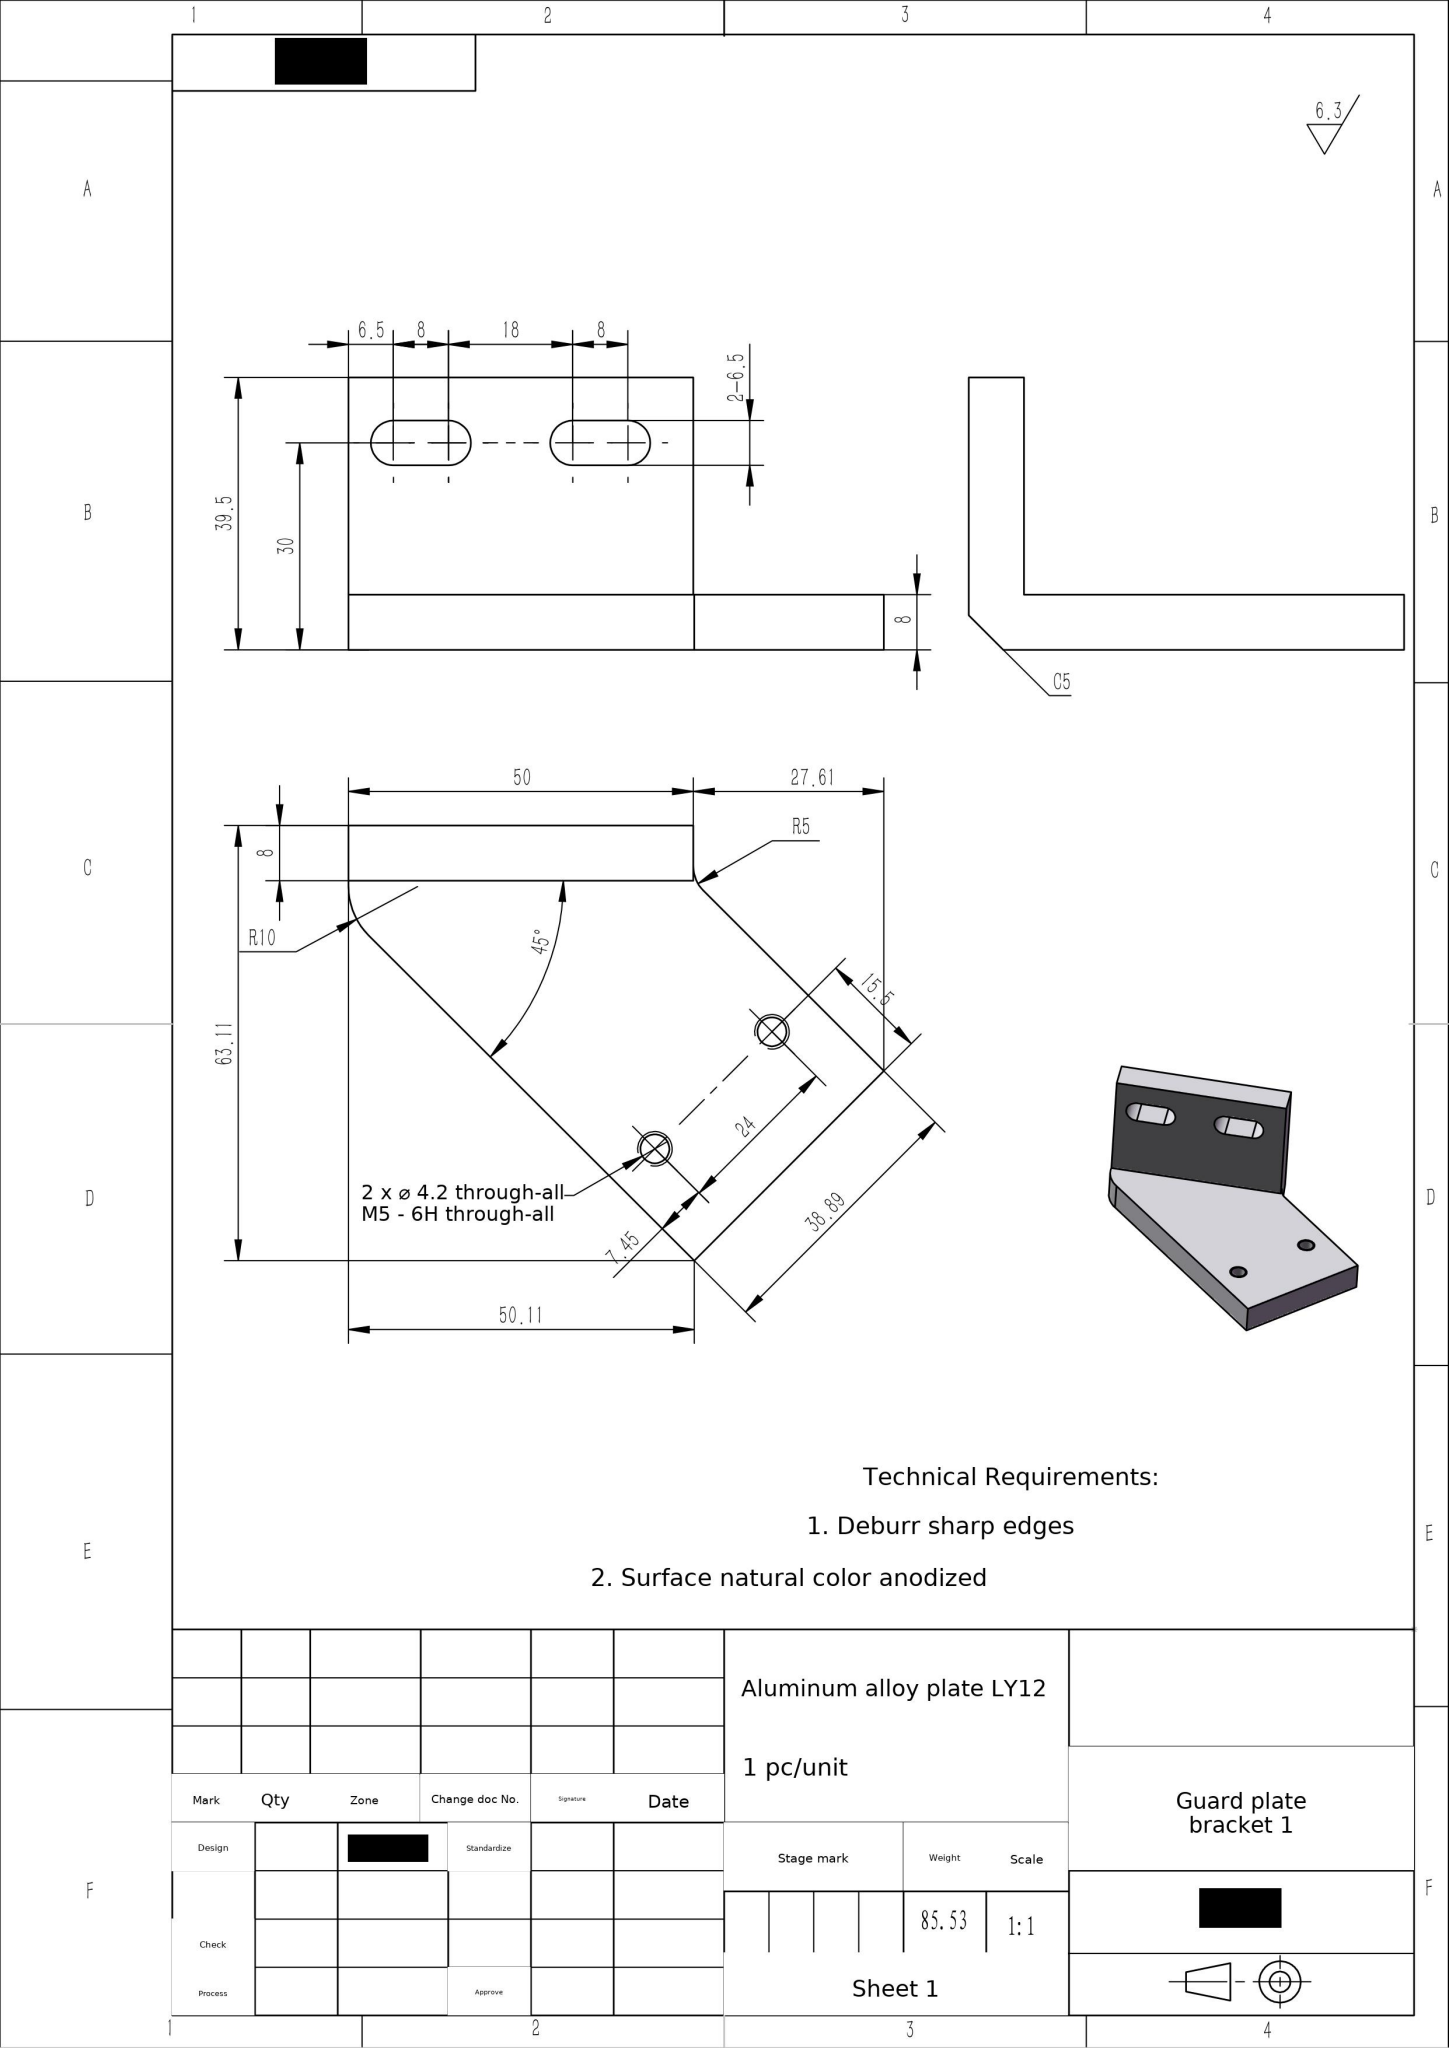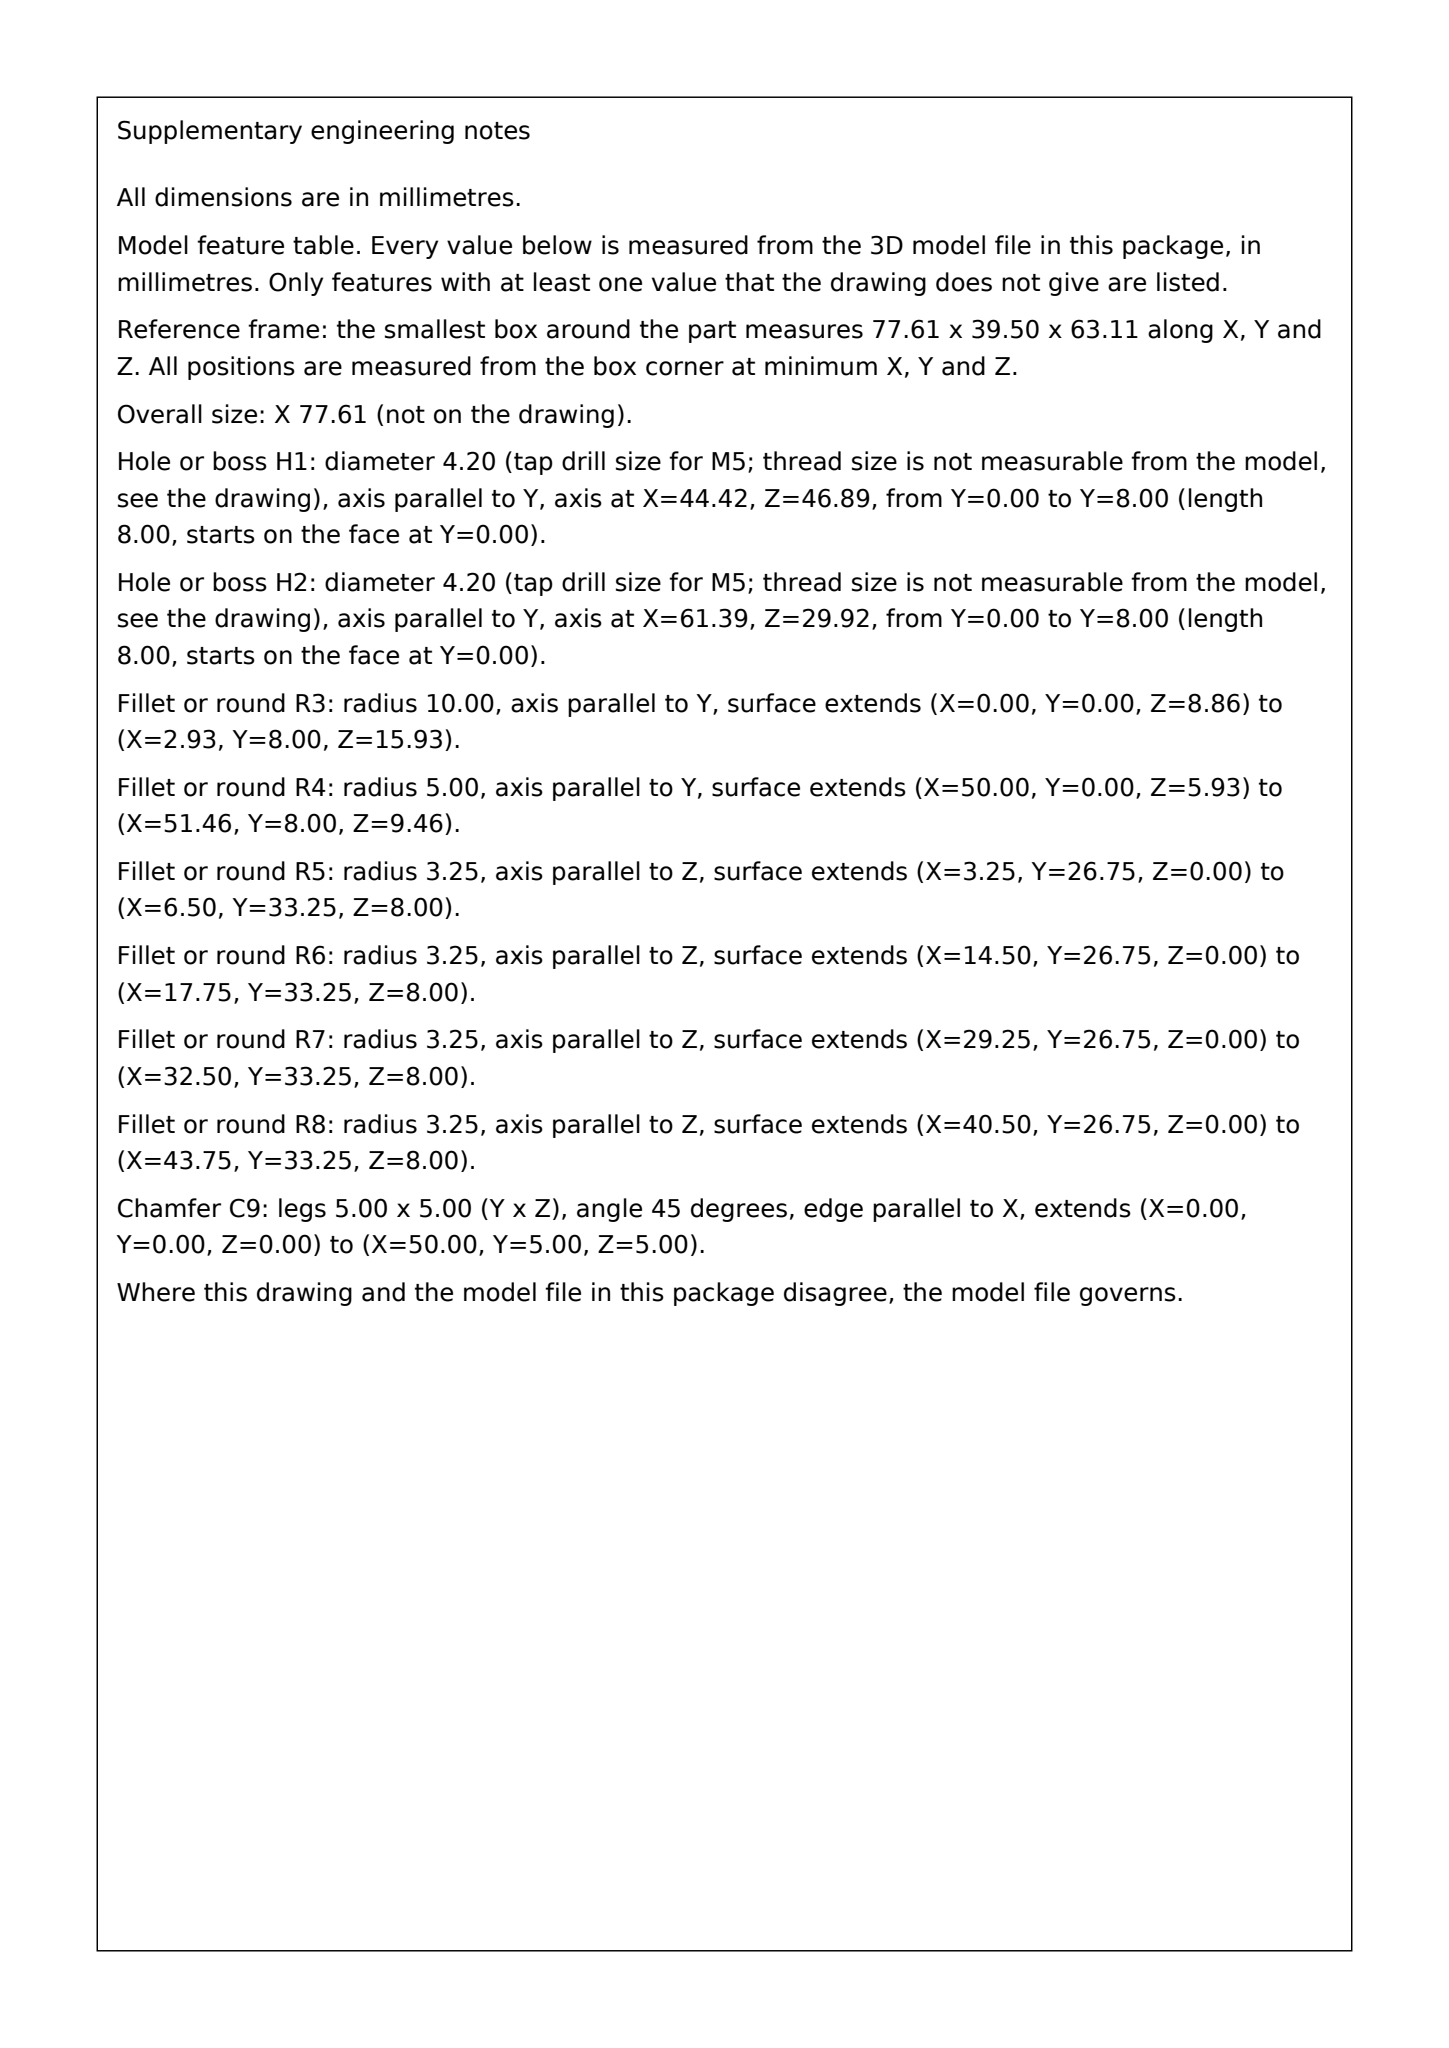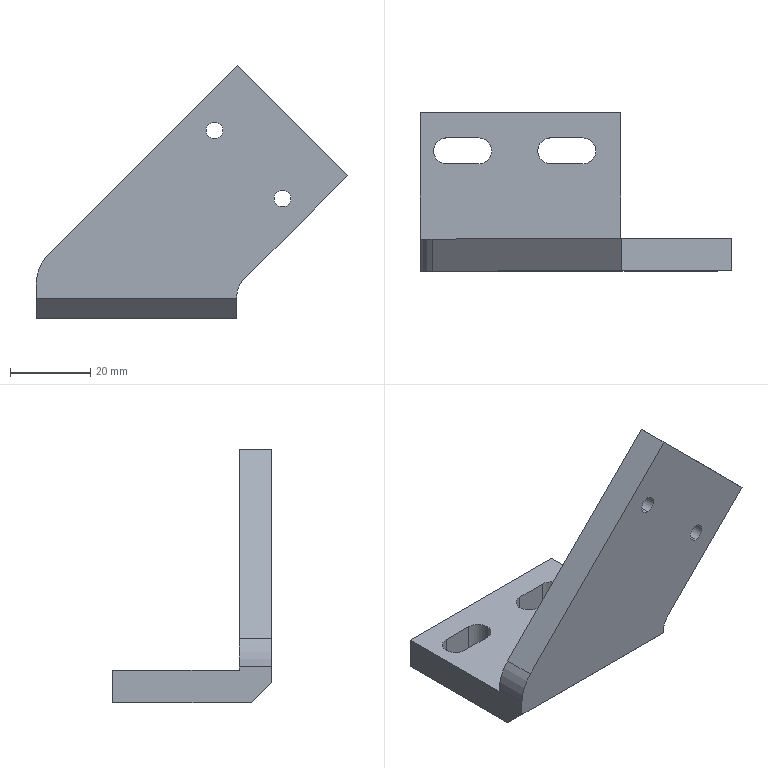Part | SolidWorks | mm | material Aluminum alloy plate LY12 | 1 solid | 27 faces | box 77.61 x 39.5 x 63.11 mm | volume 31677 mm3 | plane 15 | cylinder 12 | commonest cylinder face diameters 6.5 x6 4.2 x4 10 x1 20 x1
STEP:
#1=CARTESIAN_POINT('',(38.887,-24.,27.816));
#2=VERTEX_POINT('',#1);
#3=CARTESIAN_POINT('',(38.887,-24.,32.016));
#4=VERTEX_POINT('',#3);
#5=CARTESIAN_POINT('',(38.887,-24.,29.916));
#6=DIRECTION('',(0.,1.,0.));
#7=DIRECTION('',(0.,0.,1.));
#8=AXIS2_PLACEMENT_3D('',#5,#6,#7);
#9=CIRCLE('',#8,2.1);
#10=EDGE_CURVE('',#2,#4,#9,.T.);
#11=ORIENTED_EDGE('',*,*,#10,.F.);
#12=CARTESIAN_POINT('',(38.887,-16.,27.816));
#13=VERTEX_POINT('',#12);
#14=CARTESIAN_POINT('',(38.887,-16.,27.816));
#15=DIRECTION('',(0.,1.,0.));
#16=VECTOR('',#15,1000.);
#17=LINE('',#14,#16);
#18=EDGE_CURVE('',#2,#13,#17,.T.);
#19=ORIENTED_EDGE('',*,*,#18,.T.);
#20=CARTESIAN_POINT('',(38.887,-16.,32.016));
#21=VERTEX_POINT('',#20);
#22=CARTESIAN_POINT('',(38.887,-16.,29.916));
#23=DIRECTION('',(0.,1.,0.));
#24=DIRECTION('',(0.,0.,1.));
#25=AXIS2_PLACEMENT_3D('',#22,#23,#24);
#26=CIRCLE('',#25,2.1);
#27=EDGE_CURVE('',#13,#21,#26,.T.);
#28=ORIENTED_EDGE('',*,*,#27,.T.);
#29=CARTESIAN_POINT('',(38.887,-16.,32.016));
#30=DIRECTION('',(0.,1.,0.));
#31=VECTOR('',#30,1000.);
#32=LINE('',#29,#31);
#33=EDGE_CURVE('',#4,#21,#32,.T.);
#34=ORIENTED_EDGE('',*,*,#33,.F.);
#35=EDGE_LOOP('',(#11,#19,#28,#34));
#36=FACE_OUTER_BOUND('',#35,.T.);
#37=CARTESIAN_POINT('',(38.887,-16.,29.916));
#38=DIRECTION('',(0.,1.,0.));
#39=DIRECTION('',(0.,0.,1.));
#40=AXIS2_PLACEMENT_3D('',#37,#38,#39);
#41=CYLINDRICAL_SURFACE('',#40,2.1);
#42=ADVANCED_FACE('',(#36),#41,.F.);
#43=CARTESIAN_POINT('',(21.916,-24.,44.787));
#44=VERTEX_POINT('',#43);
#45=CARTESIAN_POINT('',(21.916,-24.,48.987));
#46=VERTEX_POINT('',#45);
#47=CARTESIAN_POINT('',(21.916,-24.,46.887));
#48=DIRECTION('',(0.,1.,0.));
#49=DIRECTION('',(0.,0.,1.));
#50=AXIS2_PLACEMENT_3D('',#47,#48,#49);
#51=CIRCLE('',#50,2.1);
#52=EDGE_CURVE('',#44,#46,#51,.T.);
#53=ORIENTED_EDGE('',*,*,#52,.F.);
#54=CARTESIAN_POINT('',(21.916,-16.,44.787));
#55=VERTEX_POINT('',#54);
#56=CARTESIAN_POINT('',(21.916,-16.,44.787));
#57=DIRECTION('',(0.,1.,0.));
#58=VECTOR('',#57,1000.);
#59=LINE('',#56,#58);
#60=EDGE_CURVE('',#44,#55,#59,.T.);
#61=ORIENTED_EDGE('',*,*,#60,.T.);
#62=CARTESIAN_POINT('',(21.916,-16.,48.987));
#63=VERTEX_POINT('',#62);
#64=CARTESIAN_POINT('',(21.916,-16.,46.887));
#65=DIRECTION('',(0.,1.,0.));
#66=DIRECTION('',(0.,0.,1.));
#67=AXIS2_PLACEMENT_3D('',#64,#65,#66);
#68=CIRCLE('',#67,2.1);
#69=EDGE_CURVE('',#55,#63,#68,.T.);
#70=ORIENTED_EDGE('',*,*,#69,.T.);
#71=CARTESIAN_POINT('',(21.916,-16.,48.987));
#72=DIRECTION('',(0.,1.,0.));
#73=VECTOR('',#72,1000.);
#74=LINE('',#71,#73);
#75=EDGE_CURVE('',#46,#63,#74,.T.);
#76=ORIENTED_EDGE('',*,*,#75,.F.);
#77=EDGE_LOOP('',(#53,#61,#70,#76));
#78=FACE_OUTER_BOUND('',#77,.T.);
#79=CARTESIAN_POINT('',(21.916,-16.,46.887));
#80=DIRECTION('',(0.,1.,0.));
#81=DIRECTION('',(0.,0.,1.));
#82=AXIS2_PLACEMENT_3D('',#79,#80,#81);
#83=CYLINDRICAL_SURFACE('',#82,2.1);
#84=ADVANCED_FACE('',(#78),#83,.F.);
#85=CARTESIAN_POINT('',(-4.75,6.,0.));
#86=VERTEX_POINT('',#85);
#87=CARTESIAN_POINT('',(-8.,9.25,0.));
#88=VERTEX_POINT('',#87);
#89=CARTESIAN_POINT('',(-8.,6.,0.));
#90=DIRECTION('',(0.,0.,1.));
#91=DIRECTION('',(1.,0.,0.));
#92=AXIS2_PLACEMENT_3D('',#89,#90,#91);
#93=CIRCLE('',#92,3.25);
#94=EDGE_CURVE('',#86,#88,#93,.T.);
#95=ORIENTED_EDGE('',*,*,#94,.F.);
#96=CARTESIAN_POINT('',(-4.75,6.,8.));
#97=VERTEX_POINT('',#96);
#98=CARTESIAN_POINT('',(-4.75,6.,0.));
#99=DIRECTION('',(0.,0.,1.));
#100=VECTOR('',#99,1000.);
#101=LINE('',#98,#100);
#102=EDGE_CURVE('',#86,#97,#101,.T.);
#103=ORIENTED_EDGE('',*,*,#102,.T.);
#104=CARTESIAN_POINT('',(-8.,9.25,8.));
#105=VERTEX_POINT('',#104);
#106=CARTESIAN_POINT('',(-8.,6.,8.));
#107=DIRECTION('',(0.,0.,1.));
#108=DIRECTION('',(1.,0.,0.));
#109=AXIS2_PLACEMENT_3D('',#106,#107,#108);
#110=CIRCLE('',#109,3.25);
#111=EDGE_CURVE('',#97,#105,#110,.T.);
#112=ORIENTED_EDGE('',*,*,#111,.T.);
#113=CARTESIAN_POINT('',(-8.,9.25,0.));
#114=DIRECTION('',(0.,0.,1.));
#115=VECTOR('',#114,1000.);
#116=LINE('',#113,#115);
#117=EDGE_CURVE('',#88,#105,#116,.T.);
#118=ORIENTED_EDGE('',*,*,#117,.F.);
#119=EDGE_LOOP('',(#95,#103,#112,#118));
#120=FACE_OUTER_BOUND('',#119,.T.);
#121=CARTESIAN_POINT('',(-8.,6.,0.));
#122=DIRECTION('',(0.,0.,1.));
#123=DIRECTION('',(1.,0.,0.));
#124=AXIS2_PLACEMENT_3D('',#121,#122,#123);
#125=CYLINDRICAL_SURFACE('',#124,3.25);
#126=ADVANCED_FACE('',(#120),#125,.F.);
#127=CARTESIAN_POINT('',(21.25,6.,0.));
#128=VERTEX_POINT('',#127);
#129=CARTESIAN_POINT('',(18.,9.25,0.));
#130=VERTEX_POINT('',#129);
#131=CARTESIAN_POINT('',(18.,6.,0.));
#132=DIRECTION('',(0.,0.,1.));
#133=DIRECTION('',(-1.,0.,0.));
#134=AXIS2_PLACEMENT_3D('',#131,#132,#133);
#135=CIRCLE('',#134,3.25);
#136=EDGE_CURVE('',#128,#130,#135,.T.);
#137=ORIENTED_EDGE('',*,*,#136,.F.);
#138=CARTESIAN_POINT('',(21.25,6.,8.));
#139=VERTEX_POINT('',#138);
#140=CARTESIAN_POINT('',(21.25,6.,0.));
#141=DIRECTION('',(0.,0.,1.));
#142=VECTOR('',#141,1000.);
#143=LINE('',#140,#142);
#144=EDGE_CURVE('',#128,#139,#143,.T.);
#145=ORIENTED_EDGE('',*,*,#144,.T.);
#146=CARTESIAN_POINT('',(18.,9.25,8.));
#147=VERTEX_POINT('',#146);
#148=CARTESIAN_POINT('',(18.,6.,8.));
#149=DIRECTION('',(0.,0.,1.));
#150=DIRECTION('',(-1.,0.,0.));
#151=AXIS2_PLACEMENT_3D('',#148,#149,#150);
#152=CIRCLE('',#151,3.25);
#153=EDGE_CURVE('',#139,#147,#152,.T.);
#154=ORIENTED_EDGE('',*,*,#153,.T.);
#155=CARTESIAN_POINT('',(18.,9.25,0.));
#156=DIRECTION('',(0.,0.,1.));
#157=VECTOR('',#156,1000.);
#158=LINE('',#155,#157);
#159=EDGE_CURVE('',#130,#147,#158,.T.);
#160=ORIENTED_EDGE('',*,*,#159,.F.);
#161=EDGE_LOOP('',(#137,#145,#154,#160));
#162=FACE_OUTER_BOUND('',#161,.T.);
#163=CARTESIAN_POINT('',(18.,6.,0.));
#164=DIRECTION('',(0.,0.,1.));
#165=DIRECTION('',(1.,0.,0.));
#166=AXIS2_PLACEMENT_3D('',#163,#164,#165);
#167=CYLINDRICAL_SURFACE('',#166,3.25);
#168=ADVANCED_FACE('',(#162),#167,.F.);
#169=CARTESIAN_POINT('',(27.5,-24.,5.929));
#170=VERTEX_POINT('',#169);
#171=CARTESIAN_POINT('',(27.5,-24.,5.));
#172=VERTEX_POINT('',#171);
#173=CARTESIAN_POINT('',(27.5,-24.,8.));
#174=DIRECTION('',(0.,0.,-1.));
#175=VECTOR('',#174,1000.);
#176=LINE('',#173,#175);
#177=EDGE_CURVE('',#170,#172,#176,.T.);
#178=ORIENTED_EDGE('',*,*,#177,.T.);
#179=CARTESIAN_POINT('',(27.5,-19.,0.));
#180=VERTEX_POINT('',#179);
#181=CARTESIAN_POINT('',(27.5,-24.,5.));
#182=DIRECTION('',(0.,0.7071,-0.7071));
#183=VECTOR('',#182,1000.);
#184=LINE('',#181,#183);
#185=EDGE_CURVE('',#172,#180,#184,.T.);
#186=ORIENTED_EDGE('',*,*,#185,.T.);
#187=CARTESIAN_POINT('',(27.5,15.5,0.));
#188=VERTEX_POINT('',#187);
#189=CARTESIAN_POINT('',(27.5,16.,0.));
#190=DIRECTION('',(0.,1.,0.));
#191=VECTOR('',#190,1000.);
#192=LINE('',#189,#191);
#193=EDGE_CURVE('',#180,#188,#192,.T.);
#194=ORIENTED_EDGE('',*,*,#193,.T.);
#195=CARTESIAN_POINT('',(27.5,15.5,8.));
#196=VERTEX_POINT('',#195);
#197=CARTESIAN_POINT('',(27.5,15.5,8.));
#198=DIRECTION('',(0.,0.,-1.));
#199=VECTOR('',#198,1000.);
#200=LINE('',#197,#199);
#201=EDGE_CURVE('',#196,#188,#200,.T.);
#202=ORIENTED_EDGE('',*,*,#201,.F.);
#203=CARTESIAN_POINT('',(27.5,-16.,8.));
#204=VERTEX_POINT('',#203);
#205=CARTESIAN_POINT('',(27.5,16.,8.));
#206=DIRECTION('',(0.,1.,0.));
#207=VECTOR('',#206,1000.);
#208=LINE('',#205,#207);
#209=EDGE_CURVE('',#204,#196,#208,.T.);
#210=ORIENTED_EDGE('',*,*,#209,.F.);
#211=CARTESIAN_POINT('',(27.5,-16.,5.929));
#212=VERTEX_POINT('',#211);
#213=CARTESIAN_POINT('',(27.5,-16.,8.));
#214=DIRECTION('',(0.,0.,-1.));
#215=VECTOR('',#214,1000.);
#216=LINE('',#213,#215);
#217=EDGE_CURVE('',#204,#212,#216,.T.);
#218=ORIENTED_EDGE('',*,*,#217,.T.);
#219=CARTESIAN_POINT('',(27.5,-16.,5.929));
#220=DIRECTION('',(0.,-1.,0.));
#221=VECTOR('',#220,1000.);
#222=LINE('',#219,#221);
#223=EDGE_CURVE('',#212,#170,#222,.T.);
#224=ORIENTED_EDGE('',*,*,#223,.T.);
#225=EDGE_LOOP('',(#178,#186,#194,#202,#210,#218,#224));
#226=FACE_OUTER_BOUND('',#225,.T.);
#227=CARTESIAN_POINT('',(27.5,16.,8.));
#228=DIRECTION('',(-1.,0.,0.));
#229=DIRECTION('',(0.,0.,1.));
#230=AXIS2_PLACEMENT_3D('',#227,#228,#229);
#231=PLANE('',#230);
#232=ADVANCED_FACE('',(#226),#231,.F.);
#233=CARTESIAN_POINT('',(-22.5,15.5,0.));
#234=VERTEX_POINT('',#233);
#235=CARTESIAN_POINT('',(-27.5,15.5,0.));
#236=DIRECTION('',(-1.,0.,0.));
#237=VECTOR('',#236,1000.);
#238=LINE('',#235,#237);
#239=EDGE_CURVE('',#188,#234,#238,.T.);
#240=ORIENTED_EDGE('',*,*,#239,.T.);
#241=CARTESIAN_POINT('',(-22.5,15.5,8.));
#242=VERTEX_POINT('',#241);
#243=CARTESIAN_POINT('',(-22.5,15.5,0.));
#244=DIRECTION('',(-0.,0.,-1.));
#245=VECTOR('',#244,1000.);
#246=LINE('',#243,#245);
#247=EDGE_CURVE('',#242,#234,#246,.T.);
#248=ORIENTED_EDGE('',*,*,#247,.F.);
#249=CARTESIAN_POINT('',(-27.5,15.5,8.));
#250=DIRECTION('',(-1.,0.,0.));
#251=VECTOR('',#250,1000.);
#252=LINE('',#249,#251);
#253=EDGE_CURVE('',#196,#242,#252,.T.);
#254=ORIENTED_EDGE('',*,*,#253,.F.);
#255=ORIENTED_EDGE('',*,*,#201,.T.);
#256=EDGE_LOOP('',(#240,#248,#254,#255));
#257=FACE_OUTER_BOUND('',#256,.T.);
#258=CARTESIAN_POINT('',(-27.5,15.5,8.));
#259=DIRECTION('',(0.,-1.,0.));
#260=DIRECTION('',(0.,0.,-1.));
#261=AXIS2_PLACEMENT_3D('',#258,#259,#260);
#262=PLANE('',#261);
#263=ADVANCED_FACE('',(#257),#262,.F.);
#264=CARTESIAN_POINT('',(38.887,-24.,29.916));
#265=DIRECTION('',(0.,1.,0.));
#266=DIRECTION('',(0.,0.,1.));
#267=AXIS2_PLACEMENT_3D('',#264,#265,#266);
#268=CIRCLE('',#267,2.1);
#269=EDGE_CURVE('',#4,#2,#268,.T.);
#270=ORIENTED_EDGE('',*,*,#269,.T.);
#271=ORIENTED_EDGE('',*,*,#10,.T.);
#272=EDGE_LOOP('',(#270,#271));
#273=FACE_BOUND('',#272,.T.);
#274=CARTESIAN_POINT('',(21.916,-24.,46.887));
#275=DIRECTION('',(0.,1.,0.));
#276=DIRECTION('',(0.,0.,1.));
#277=AXIS2_PLACEMENT_3D('',#274,#275,#276);
#278=CIRCLE('',#277,2.1);
#279=EDGE_CURVE('',#46,#44,#278,.T.);
#280=ORIENTED_EDGE('',*,*,#279,.T.);
#281=ORIENTED_EDGE('',*,*,#52,.T.);
#282=EDGE_LOOP('',(#280,#281));
#283=FACE_BOUND('',#282,.T.);
#284=CARTESIAN_POINT('',(-22.5,-24.,8.858));
#285=VERTEX_POINT('',#284);
#286=CARTESIAN_POINT('',(-22.5,-24.,5.));
#287=VERTEX_POINT('',#286);
#288=CARTESIAN_POINT('',(-22.5,-24.,0.));
#289=DIRECTION('',(-0.,0.,-1.));
#290=VECTOR('',#289,1000.);
#291=LINE('',#288,#290);
#292=EDGE_CURVE('',#285,#287,#291,.T.);
#293=ORIENTED_EDGE('',*,*,#292,.T.);
#294=CARTESIAN_POINT('',(-27.5,-24.,5.));
#295=DIRECTION('',(1.,0.,0.));
#296=VECTOR('',#295,1000.);
#297=LINE('',#294,#296);
#298=EDGE_CURVE('',#287,#172,#297,.T.);
#299=ORIENTED_EDGE('',*,*,#298,.T.);
#300=ORIENTED_EDGE('',*,*,#177,.F.);
#301=CARTESIAN_POINT('',(28.964,-24.,9.464));
#302=VERTEX_POINT('',#301);
#303=CARTESIAN_POINT('',(32.5,-24.,5.929));
#304=DIRECTION('',(0.,1.,0.));
#305=DIRECTION('',(0.,0.,1.));
#306=AXIS2_PLACEMENT_3D('',#303,#304,#305);
#307=CIRCLE('',#306,5.);
#308=EDGE_CURVE('',#170,#302,#307,.T.);
#309=ORIENTED_EDGE('',*,*,#308,.T.);
#310=CARTESIAN_POINT('',(55.112,-24.,35.612));
#311=VERTEX_POINT('',#310);
#312=CARTESIAN_POINT('',(27.5,-24.,8.));
#313=DIRECTION('',(-0.7071,0.,-0.7071));
#314=VECTOR('',#313,1000.);
#315=LINE('',#312,#314);
#316=EDGE_CURVE('',#311,#302,#315,.T.);
#317=ORIENTED_EDGE('',*,*,#316,.F.);
#318=CARTESIAN_POINT('',(27.612,-24.,63.112));
#319=VERTEX_POINT('',#318);
#320=CARTESIAN_POINT('',(55.112,-24.,35.612));
#321=DIRECTION('',(-0.7071,0.,0.7071));
#322=VECTOR('',#321,1000.);
#323=LINE('',#320,#322);
#324=EDGE_CURVE('',#311,#319,#323,.T.);
#325=ORIENTED_EDGE('',*,*,#324,.T.);
#326=CARTESIAN_POINT('',(-19.571,-24.,15.929));
#327=VERTEX_POINT('',#326);
#328=CARTESIAN_POINT('',(-27.5,-24.,8.));
#329=DIRECTION('',(0.7071,0.,0.7071));
#330=VECTOR('',#329,1000.);
#331=LINE('',#328,#330);
#332=EDGE_CURVE('',#327,#319,#331,.T.);
#333=ORIENTED_EDGE('',*,*,#332,.F.);
#334=CARTESIAN_POINT('',(-12.5,-24.,8.858));
#335=DIRECTION('',(0.,-1.,0.));
#336=DIRECTION('',(0.,0.,1.));
#337=AXIS2_PLACEMENT_3D('',#334,#335,#336);
#338=CIRCLE('',#337,10.);
#339=EDGE_CURVE('',#327,#285,#338,.T.);
#340=ORIENTED_EDGE('',*,*,#339,.T.);
#341=EDGE_LOOP('',(#293,#299,#300,#309,#317,#325,#333,#340));
#342=FACE_OUTER_BOUND('',#341,.T.);
#343=CARTESIAN_POINT('',(-27.5,-24.,8.));
#344=DIRECTION('',(0.,1.,0.));
#345=DIRECTION('',(0.,0.,1.));
#346=AXIS2_PLACEMENT_3D('',#343,#344,#345);
#347=PLANE('',#346);
#348=ADVANCED_FACE('',(#273,#283,#342),#347,.F.);
#349=CARTESIAN_POINT('',(-22.5,-16.,8.));
#350=VERTEX_POINT('',#349);
#351=CARTESIAN_POINT('',(-22.5,0.,8.));
#352=DIRECTION('',(0.,1.,0.));
#353=VECTOR('',#352,1000.);
#354=LINE('',#351,#353);
#355=EDGE_CURVE('',#350,#242,#354,.T.);
#356=ORIENTED_EDGE('',*,*,#355,.F.);
#357=CARTESIAN_POINT('',(27.5,-16.,8.));
#358=DIRECTION('',(-1.,0.,0.));
#359=VECTOR('',#358,1000.);
#360=LINE('',#357,#359);
#361=EDGE_CURVE('',#204,#350,#360,.T.);
#362=ORIENTED_EDGE('',*,*,#361,.F.);
#363=ORIENTED_EDGE('',*,*,#209,.T.);
#364=ORIENTED_EDGE('',*,*,#253,.T.);
#365=EDGE_LOOP('',(#356,#362,#363,#364));
#366=FACE_OUTER_BOUND('',#365,.T.);
#367=CARTESIAN_POINT('',(-16.,9.25,8.));
#368=VERTEX_POINT('',#367);
#369=CARTESIAN_POINT('',(-16.,2.75,8.));
#370=VERTEX_POINT('',#369);
#371=CARTESIAN_POINT('',(-16.,6.,8.));
#372=DIRECTION('',(0.,0.,1.));
#373=DIRECTION('',(1.,0.,0.));
#374=AXIS2_PLACEMENT_3D('',#371,#372,#373);
#375=CIRCLE('',#374,3.25);
#376=EDGE_CURVE('',#368,#370,#375,.T.);
#377=ORIENTED_EDGE('',*,*,#376,.F.);
#378=CARTESIAN_POINT('',(-16.,9.25,8.));
#379=DIRECTION('',(-1.,-0.,0.));
#380=VECTOR('',#379,1000.);
#381=LINE('',#378,#380);
#382=EDGE_CURVE('',#105,#368,#381,.T.);
#383=ORIENTED_EDGE('',*,*,#382,.F.);
#384=ORIENTED_EDGE('',*,*,#111,.F.);
#385=CARTESIAN_POINT('',(-8.,2.75,8.));
#386=VERTEX_POINT('',#385);
#387=CARTESIAN_POINT('',(-8.,6.,8.));
#388=DIRECTION('',(0.,0.,1.));
#389=DIRECTION('',(1.,0.,0.));
#390=AXIS2_PLACEMENT_3D('',#387,#388,#389);
#391=CIRCLE('',#390,3.25);
#392=EDGE_CURVE('',#386,#97,#391,.T.);
#393=ORIENTED_EDGE('',*,*,#392,.F.);
#394=CARTESIAN_POINT('',(-16.,2.75,8.));
#395=DIRECTION('',(1.,0.,0.));
#396=VECTOR('',#395,1000.);
#397=LINE('',#394,#396);
#398=EDGE_CURVE('',#370,#386,#397,.T.);
#399=ORIENTED_EDGE('',*,*,#398,.F.);
#400=EDGE_LOOP('',(#377,#383,#384,#393,#399));
#401=FACE_BOUND('',#400,.T.);
#402=CARTESIAN_POINT('',(18.,2.75,8.));
#403=VERTEX_POINT('',#402);
#404=CARTESIAN_POINT('',(18.,6.,8.));
#405=DIRECTION('',(0.,0.,1.));
#406=DIRECTION('',(-1.,0.,0.));
#407=AXIS2_PLACEMENT_3D('',#404,#405,#406);
#408=CIRCLE('',#407,3.25);
#409=EDGE_CURVE('',#403,#139,#408,.T.);
#410=ORIENTED_EDGE('',*,*,#409,.F.);
#411=CARTESIAN_POINT('',(10.,2.75,8.));
#412=VERTEX_POINT('',#411);
#413=CARTESIAN_POINT('',(18.,2.75,8.));
#414=DIRECTION('',(1.,0.,0.));
#415=VECTOR('',#414,1000.);
#416=LINE('',#413,#415);
#417=EDGE_CURVE('',#412,#403,#416,.T.);
#418=ORIENTED_EDGE('',*,*,#417,.F.);
#419=CARTESIAN_POINT('',(10.,9.25,8.));
#420=VERTEX_POINT('',#419);
#421=CARTESIAN_POINT('',(10.,6.,8.));
#422=DIRECTION('',(0.,0.,1.));
#423=DIRECTION('',(-1.,0.,0.));
#424=AXIS2_PLACEMENT_3D('',#421,#422,#423);
#425=CIRCLE('',#424,3.25);
#426=EDGE_CURVE('',#420,#412,#425,.T.);
#427=ORIENTED_EDGE('',*,*,#426,.F.);
#428=CARTESIAN_POINT('',(18.,9.25,8.));
#429=DIRECTION('',(-1.,0.,0.));
#430=VECTOR('',#429,1000.);
#431=LINE('',#428,#430);
#432=EDGE_CURVE('',#147,#420,#431,.T.);
#433=ORIENTED_EDGE('',*,*,#432,.F.);
#434=ORIENTED_EDGE('',*,*,#153,.F.);
#435=EDGE_LOOP('',(#410,#418,#427,#433,#434));
#436=FACE_BOUND('',#435,.T.);
#437=CARTESIAN_POINT('',(0.,0.,8.));
#438=DIRECTION('',(0.,0.,1.));
#439=DIRECTION('',(1.,0.,0.));
#440=AXIS2_PLACEMENT_3D('',#437,#438,#439);
#441=PLANE('',#440);
#442=ADVANCED_FACE('',(#366,#401,#436),#441,.T.);
#443=CARTESIAN_POINT('',(-16.,9.25,0.));
#444=VERTEX_POINT('',#443);
#445=CARTESIAN_POINT('',(-16.,9.25,0.));
#446=DIRECTION('',(-1.,-0.,0.));
#447=VECTOR('',#446,1000.);
#448=LINE('',#445,#447);
#449=EDGE_CURVE('',#88,#444,#448,.T.);
#450=ORIENTED_EDGE('',*,*,#449,.T.);
#451=CARTESIAN_POINT('',(-16.,2.75,0.));
#452=VERTEX_POINT('',#451);
#453=CARTESIAN_POINT('',(-16.,6.,0.));
#454=DIRECTION('',(0.,0.,1.));
#455=DIRECTION('',(1.,0.,0.));
#456=AXIS2_PLACEMENT_3D('',#453,#454,#455);
#457=CIRCLE('',#456,3.25);
#458=EDGE_CURVE('',#444,#452,#457,.T.);
#459=ORIENTED_EDGE('',*,*,#458,.T.);
#460=CARTESIAN_POINT('',(-8.,2.75,0.));
#461=VERTEX_POINT('',#460);
#462=CARTESIAN_POINT('',(-16.,2.75,0.));
#463=DIRECTION('',(1.,0.,0.));
#464=VECTOR('',#463,1000.);
#465=LINE('',#462,#464);
#466=EDGE_CURVE('',#452,#461,#465,.T.);
#467=ORIENTED_EDGE('',*,*,#466,.T.);
#468=CARTESIAN_POINT('',(-8.,6.,0.));
#469=DIRECTION('',(0.,0.,1.));
#470=DIRECTION('',(1.,0.,0.));
#471=AXIS2_PLACEMENT_3D('',#468,#469,#470);
#472=CIRCLE('',#471,3.25);
#473=EDGE_CURVE('',#461,#86,#472,.T.);
#474=ORIENTED_EDGE('',*,*,#473,.T.);
#475=ORIENTED_EDGE('',*,*,#94,.T.);
#476=EDGE_LOOP('',(#450,#459,#467,#474,#475));
#477=FACE_BOUND('',#476,.T.);
#478=CARTESIAN_POINT('',(10.,2.75,0.));
#479=VERTEX_POINT('',#478);
#480=CARTESIAN_POINT('',(18.,2.75,0.));
#481=VERTEX_POINT('',#480);
#482=CARTESIAN_POINT('',(18.,2.75,0.));
#483=DIRECTION('',(1.,0.,0.));
#484=VECTOR('',#483,1000.);
#485=LINE('',#482,#484);
#486=EDGE_CURVE('',#479,#481,#485,.T.);
#487=ORIENTED_EDGE('',*,*,#486,.T.);
#488=CARTESIAN_POINT('',(18.,6.,0.));
#489=DIRECTION('',(0.,0.,1.));
#490=DIRECTION('',(-1.,0.,0.));
#491=AXIS2_PLACEMENT_3D('',#488,#489,#490);
#492=CIRCLE('',#491,3.25);
#493=EDGE_CURVE('',#481,#128,#492,.T.);
#494=ORIENTED_EDGE('',*,*,#493,.T.);
#495=ORIENTED_EDGE('',*,*,#136,.T.);
#496=CARTESIAN_POINT('',(10.,9.25,0.));
#497=VERTEX_POINT('',#496);
#498=CARTESIAN_POINT('',(18.,9.25,0.));
#499=DIRECTION('',(-1.,0.,0.));
#500=VECTOR('',#499,1000.);
#501=LINE('',#498,#500);
#502=EDGE_CURVE('',#130,#497,#501,.T.);
#503=ORIENTED_EDGE('',*,*,#502,.T.);
#504=CARTESIAN_POINT('',(10.,6.,0.));
#505=DIRECTION('',(0.,0.,1.));
#506=DIRECTION('',(-1.,0.,0.));
#507=AXIS2_PLACEMENT_3D('',#504,#505,#506);
#508=CIRCLE('',#507,3.25);
#509=EDGE_CURVE('',#497,#479,#508,.T.);
#510=ORIENTED_EDGE('',*,*,#509,.T.);
#511=EDGE_LOOP('',(#487,#494,#495,#503,#510));
#512=FACE_BOUND('',#511,.T.);
#513=ORIENTED_EDGE('',*,*,#193,.F.);
#514=CARTESIAN_POINT('',(-22.5,-19.,0.));
#515=VERTEX_POINT('',#514);
#516=CARTESIAN_POINT('',(0.,-19.,0.));
#517=DIRECTION('',(-1.,0.,0.));
#518=VECTOR('',#517,1000.);
#519=LINE('',#516,#518);
#520=EDGE_CURVE('',#180,#515,#519,.T.);
#521=ORIENTED_EDGE('',*,*,#520,.T.);
#522=CARTESIAN_POINT('',(-22.5,-24.,0.));
#523=DIRECTION('',(0.,1.,0.));
#524=VECTOR('',#523,1000.);
#525=LINE('',#522,#524);
#526=EDGE_CURVE('',#515,#234,#525,.T.);
#527=ORIENTED_EDGE('',*,*,#526,.T.);
#528=ORIENTED_EDGE('',*,*,#239,.F.);
#529=EDGE_LOOP('',(#513,#521,#527,#528));
#530=FACE_OUTER_BOUND('',#529,.T.);
#531=CARTESIAN_POINT('',(0.,0.,0.));
#532=DIRECTION('',(0.,0.,1.));
#533=DIRECTION('',(1.,0.,0.));
#534=AXIS2_PLACEMENT_3D('',#531,#532,#533);
#535=PLANE('',#534);
#536=ADVANCED_FACE('',(#477,#512,#530),#535,.F.);
#537=CARTESIAN_POINT('',(-19.571,-16.,15.929));
#538=VERTEX_POINT('',#537);
#539=CARTESIAN_POINT('',(27.612,-16.,63.112));
#540=VERTEX_POINT('',#539);
#541=CARTESIAN_POINT('',(-27.5,-16.,8.));
#542=DIRECTION('',(0.7071,0.,0.7071));
#543=VECTOR('',#542,1000.);
#544=LINE('',#541,#543);
#545=EDGE_CURVE('',#538,#540,#544,.T.);
#546=ORIENTED_EDGE('',*,*,#545,.F.);
#547=CARTESIAN_POINT('',(-19.571,-8.,15.929));
#548=DIRECTION('',(0.,-1.,0.));
#549=VECTOR('',#548,1000.);
#550=LINE('',#547,#549);
#551=EDGE_CURVE('',#538,#327,#550,.T.);
#552=ORIENTED_EDGE('',*,*,#551,.T.);
#553=ORIENTED_EDGE('',*,*,#332,.T.);
#554=CARTESIAN_POINT('',(27.612,-16.,63.112));
#555=DIRECTION('',(0.,1.,0.));
#556=VECTOR('',#555,1000.);
#557=LINE('',#554,#556);
#558=EDGE_CURVE('',#319,#540,#557,.T.);
#559=ORIENTED_EDGE('',*,*,#558,.T.);
#560=EDGE_LOOP('',(#546,#552,#553,#559));
#561=FACE_OUTER_BOUND('',#560,.T.);
#562=CARTESIAN_POINT('',(-27.5,-8.,8.));
#563=DIRECTION('',(0.7071,0.,-0.7071));
#564=DIRECTION('',(-0.7071,0.,-0.7071));
#565=AXIS2_PLACEMENT_3D('',#562,#563,#564);
#566=PLANE('',#565);
#567=ADVANCED_FACE('',(#561),#566,.F.);
#568=CARTESIAN_POINT('',(55.112,-16.,35.612));
#569=VERTEX_POINT('',#568);
#570=CARTESIAN_POINT('',(28.964,-16.,9.464));
#571=VERTEX_POINT('',#570);
#572=CARTESIAN_POINT('',(27.5,-16.,8.));
#573=DIRECTION('',(-0.7071,0.,-0.7071));
#574=VECTOR('',#573,1000.);
#575=LINE('',#572,#574);
#576=EDGE_CURVE('',#569,#571,#575,.T.);
#577=ORIENTED_EDGE('',*,*,#576,.F.);
#578=CARTESIAN_POINT('',(55.112,-16.,35.612));
#579=DIRECTION('',(0.,1.,0.));
#580=VECTOR('',#579,1000.);
#581=LINE('',#578,#580);
#582=EDGE_CURVE('',#311,#569,#581,.T.);
#583=ORIENTED_EDGE('',*,*,#582,.F.);
#584=ORIENTED_EDGE('',*,*,#316,.T.);
#585=CARTESIAN_POINT('',(28.964,-8.,9.464));
#586=DIRECTION('',(0.,1.,0.));
#587=VECTOR('',#586,1000.);
#588=LINE('',#585,#587);
#589=EDGE_CURVE('',#302,#571,#588,.T.);
#590=ORIENTED_EDGE('',*,*,#589,.T.);
#591=EDGE_LOOP('',(#577,#583,#584,#590));
#592=FACE_OUTER_BOUND('',#591,.T.);
#593=CARTESIAN_POINT('',(27.5,-8.,8.));
#594=DIRECTION('',(-0.7071,0.,0.7071));
#595=DIRECTION('',(0.7071,0.,0.7071));
#596=AXIS2_PLACEMENT_3D('',#593,#594,#595);
#597=PLANE('',#596);
#598=ADVANCED_FACE('',(#592),#597,.F.);
#599=CARTESIAN_POINT('',(-22.5,-16.,8.858));
#600=VERTEX_POINT('',#599);
#601=CARTESIAN_POINT('',(-22.5,-16.,0.));
#602=DIRECTION('',(-0.,0.,-1.));
#603=VECTOR('',#602,1000.);
#604=LINE('',#601,#603);
#605=EDGE_CURVE('',#600,#350,#604,.T.);
#606=ORIENTED_EDGE('',*,*,#605,.F.);
#607=CARTESIAN_POINT('',(-12.5,-16.,8.858));
#608=DIRECTION('',(0.,1.,0.));
#609=DIRECTION('',(0.,0.,1.));
#610=AXIS2_PLACEMENT_3D('',#607,#608,#609);
#611=CIRCLE('',#610,10.);
#612=EDGE_CURVE('',#600,#538,#611,.T.);
#613=ORIENTED_EDGE('',*,*,#612,.T.);
#614=ORIENTED_EDGE('',*,*,#545,.T.);
#615=CARTESIAN_POINT('',(45.362,-16.,45.362));
#616=DIRECTION('',(-0.7071,0.,0.7071));
#617=VECTOR('',#616,1000.);
#618=LINE('',#615,#617);
#619=EDGE_CURVE('',#569,#540,#618,.T.);
#620=ORIENTED_EDGE('',*,*,#619,.F.);
#621=ORIENTED_EDGE('',*,*,#576,.T.);
#622=CARTESIAN_POINT('',(32.5,-16.,5.929));
#623=DIRECTION('',(0.,-1.,0.));
#624=DIRECTION('',(0.,0.,1.));
#625=AXIS2_PLACEMENT_3D('',#622,#623,#624);
#626=CIRCLE('',#625,5.);
#627=EDGE_CURVE('',#571,#212,#626,.T.);
#628=ORIENTED_EDGE('',*,*,#627,.T.);
#629=ORIENTED_EDGE('',*,*,#217,.F.);
#630=ORIENTED_EDGE('',*,*,#361,.T.);
#631=EDGE_LOOP('',(#606,#613,#614,#620,#621,#628,#629,#630));
#632=FACE_OUTER_BOUND('',#631,.T.);
#633=CARTESIAN_POINT('',(38.887,-16.,29.916));
#634=DIRECTION('',(0.,1.,0.));
#635=DIRECTION('',(0.,0.,1.));
#636=AXIS2_PLACEMENT_3D('',#633,#634,#635);
#637=CIRCLE('',#636,2.1);
#638=EDGE_CURVE('',#21,#13,#637,.T.);
#639=ORIENTED_EDGE('',*,*,#638,.F.);
#640=ORIENTED_EDGE('',*,*,#27,.F.);
#641=EDGE_LOOP('',(#639,#640));
#642=FACE_BOUND('',#641,.T.);
#643=CARTESIAN_POINT('',(21.916,-16.,46.887));
#644=DIRECTION('',(0.,1.,0.));
#645=DIRECTION('',(0.,0.,1.));
#646=AXIS2_PLACEMENT_3D('',#643,#644,#645);
#647=CIRCLE('',#646,2.1);
#648=EDGE_CURVE('',#63,#55,#647,.T.);
#649=ORIENTED_EDGE('',*,*,#648,.F.);
#650=ORIENTED_EDGE('',*,*,#69,.F.);
#651=EDGE_LOOP('',(#649,#650));
#652=FACE_BOUND('',#651,.T.);
#653=CARTESIAN_POINT('',(0.,-16.,0.));
#654=DIRECTION('',(0.,1.,0.));
#655=DIRECTION('',(0.,0.,1.));
#656=AXIS2_PLACEMENT_3D('',#653,#654,#655);
#657=PLANE('',#656);
#658=ADVANCED_FACE('',(#632,#642,#652),#657,.T.);
#659=ORIENTED_EDGE('',*,*,#144,.F.);
#660=ORIENTED_EDGE('',*,*,#493,.F.);
#661=CARTESIAN_POINT('',(18.,2.75,0.));
#662=DIRECTION('',(0.,0.,1.));
#663=VECTOR('',#662,1000.);
#664=LINE('',#661,#663);
#665=EDGE_CURVE('',#481,#403,#664,.T.);
#666=ORIENTED_EDGE('',*,*,#665,.T.);
#667=ORIENTED_EDGE('',*,*,#409,.T.);
#668=EDGE_LOOP('',(#659,#660,#666,#667));
#669=FACE_OUTER_BOUND('',#668,.T.);
#670=CARTESIAN_POINT('',(18.,6.,0.));
#671=DIRECTION('',(0.,0.,1.));
#672=DIRECTION('',(1.,0.,0.));
#673=AXIS2_PLACEMENT_3D('',#670,#671,#672);
#674=CYLINDRICAL_SURFACE('',#673,3.25);
#675=ADVANCED_FACE('',(#669),#674,.F.);
#676=ORIENTED_EDGE('',*,*,#417,.T.);
#677=ORIENTED_EDGE('',*,*,#665,.F.);
#678=ORIENTED_EDGE('',*,*,#486,.F.);
#679=CARTESIAN_POINT('',(10.,2.75,0.));
#680=DIRECTION('',(0.,0.,1.));
#681=VECTOR('',#680,1000.);
#682=LINE('',#679,#681);
#683=EDGE_CURVE('',#479,#412,#682,.T.);
#684=ORIENTED_EDGE('',*,*,#683,.T.);
#685=EDGE_LOOP('',(#676,#677,#678,#684));
#686=FACE_OUTER_BOUND('',#685,.T.);
#687=CARTESIAN_POINT('',(18.,2.75,0.));
#688=DIRECTION('',(0.,-1.,0.));
#689=DIRECTION('',(0.,0.,-1.));
#690=AXIS2_PLACEMENT_3D('',#687,#688,#689);
#691=PLANE('',#690);
#692=ADVANCED_FACE('',(#686),#691,.F.);
#693=ORIENTED_EDGE('',*,*,#426,.T.);
#694=ORIENTED_EDGE('',*,*,#683,.F.);
#695=ORIENTED_EDGE('',*,*,#509,.F.);
#696=CARTESIAN_POINT('',(10.,9.25,0.));
#697=DIRECTION('',(0.,0.,1.));
#698=VECTOR('',#697,1000.);
#699=LINE('',#696,#698);
#700=EDGE_CURVE('',#497,#420,#699,.T.);
#701=ORIENTED_EDGE('',*,*,#700,.T.);
#702=EDGE_LOOP('',(#693,#694,#695,#701));
#703=FACE_OUTER_BOUND('',#702,.T.);
#704=CARTESIAN_POINT('',(10.,6.,0.));
#705=DIRECTION('',(0.,0.,1.));
#706=DIRECTION('',(1.,0.,0.));
#707=AXIS2_PLACEMENT_3D('',#704,#705,#706);
#708=CYLINDRICAL_SURFACE('',#707,3.25);
#709=ADVANCED_FACE('',(#703),#708,.F.);
#710=ORIENTED_EDGE('',*,*,#432,.T.);
#711=ORIENTED_EDGE('',*,*,#700,.F.);
#712=ORIENTED_EDGE('',*,*,#502,.F.);
#713=ORIENTED_EDGE('',*,*,#159,.T.);
#714=EDGE_LOOP('',(#710,#711,#712,#713));
#715=FACE_OUTER_BOUND('',#714,.T.);
#716=CARTESIAN_POINT('',(18.,9.25,0.));
#717=DIRECTION('',(0.,1.,0.));
#718=DIRECTION('',(-1.,0.,0.));
#719=AXIS2_PLACEMENT_3D('',#716,#717,#718);
#720=PLANE('',#719);
#721=ADVANCED_FACE('',(#715),#720,.F.);
#722=ORIENTED_EDGE('',*,*,#376,.T.);
#723=CARTESIAN_POINT('',(-16.,2.75,0.));
#724=DIRECTION('',(0.,0.,1.));
#725=VECTOR('',#724,1000.);
#726=LINE('',#723,#725);
#727=EDGE_CURVE('',#452,#370,#726,.T.);
#728=ORIENTED_EDGE('',*,*,#727,.F.);
#729=ORIENTED_EDGE('',*,*,#458,.F.);
#730=CARTESIAN_POINT('',(-16.,9.25,0.));
#731=DIRECTION('',(0.,0.,1.));
#732=VECTOR('',#731,1000.);
#733=LINE('',#730,#732);
#734=EDGE_CURVE('',#444,#368,#733,.T.);
#735=ORIENTED_EDGE('',*,*,#734,.T.);
#736=EDGE_LOOP('',(#722,#728,#729,#735));
#737=FACE_OUTER_BOUND('',#736,.T.);
#738=CARTESIAN_POINT('',(-16.,6.,0.));
#739=DIRECTION('',(0.,0.,1.));
#740=DIRECTION('',(1.,0.,0.));
#741=AXIS2_PLACEMENT_3D('',#738,#739,#740);
#742=CYLINDRICAL_SURFACE('',#741,3.25);
#743=ADVANCED_FACE('',(#737),#742,.F.);
#744=ORIENTED_EDGE('',*,*,#382,.T.);
#745=ORIENTED_EDGE('',*,*,#734,.F.);
#746=ORIENTED_EDGE('',*,*,#449,.F.);
#747=ORIENTED_EDGE('',*,*,#117,.T.);
#748=EDGE_LOOP('',(#744,#745,#746,#747));
#749=FACE_OUTER_BOUND('',#748,.T.);
#750=CARTESIAN_POINT('',(-16.,9.25,0.));
#751=DIRECTION('',(-0.,1.,0.));
#752=DIRECTION('',(-1.,-0.,0.));
#753=AXIS2_PLACEMENT_3D('',#750,#751,#752);
#754=PLANE('',#753);
#755=ADVANCED_FACE('',(#749),#754,.F.);
#756=ORIENTED_EDGE('',*,*,#102,.F.);
#757=ORIENTED_EDGE('',*,*,#473,.F.);
#758=CARTESIAN_POINT('',(-8.,2.75,0.));
#759=DIRECTION('',(0.,0.,1.));
#760=VECTOR('',#759,1000.);
#761=LINE('',#758,#760);
#762=EDGE_CURVE('',#461,#386,#761,.T.);
#763=ORIENTED_EDGE('',*,*,#762,.T.);
#764=ORIENTED_EDGE('',*,*,#392,.T.);
#765=EDGE_LOOP('',(#756,#757,#763,#764));
#766=FACE_OUTER_BOUND('',#765,.T.);
#767=CARTESIAN_POINT('',(-8.,6.,0.));
#768=DIRECTION('',(0.,0.,1.));
#769=DIRECTION('',(1.,0.,0.));
#770=AXIS2_PLACEMENT_3D('',#767,#768,#769);
#771=CYLINDRICAL_SURFACE('',#770,3.25);
#772=ADVANCED_FACE('',(#766),#771,.F.);
#773=ORIENTED_EDGE('',*,*,#398,.T.);
#774=ORIENTED_EDGE('',*,*,#762,.F.);
#775=ORIENTED_EDGE('',*,*,#466,.F.);
#776=ORIENTED_EDGE('',*,*,#727,.T.);
#777=EDGE_LOOP('',(#773,#774,#775,#776));
#778=FACE_OUTER_BOUND('',#777,.T.);
#779=CARTESIAN_POINT('',(-16.,2.75,0.));
#780=DIRECTION('',(0.,-1.,0.));
#781=DIRECTION('',(1.,0.,0.));
#782=AXIS2_PLACEMENT_3D('',#779,#780,#781);
#783=PLANE('',#782);
#784=ADVANCED_FACE('',(#778),#783,.F.);
#785=ORIENTED_EDGE('',*,*,#308,.F.);
#786=ORIENTED_EDGE('',*,*,#223,.F.);
#787=ORIENTED_EDGE('',*,*,#627,.F.);
#788=ORIENTED_EDGE('',*,*,#589,.F.);
#789=EDGE_LOOP('',(#785,#786,#787,#788));
#790=FACE_OUTER_BOUND('',#789,.T.);
#791=CARTESIAN_POINT('',(32.5,-8.,5.929));
#792=DIRECTION('',(0.,-1.,0.));
#793=DIRECTION('',(0.,0.,-1.));
#794=AXIS2_PLACEMENT_3D('',#791,#792,#793);
#795=CYLINDRICAL_SURFACE('',#794,5.);
#796=ADVANCED_FACE('',(#790),#795,.F.);
#797=ORIENTED_EDGE('',*,*,#619,.T.);
#798=ORIENTED_EDGE('',*,*,#558,.F.);
#799=ORIENTED_EDGE('',*,*,#324,.F.);
#800=ORIENTED_EDGE('',*,*,#582,.T.);
#801=EDGE_LOOP('',(#797,#798,#799,#800));
#802=FACE_OUTER_BOUND('',#801,.T.);
#803=CARTESIAN_POINT('',(55.112,-16.,35.612));
#804=DIRECTION('',(-0.7071,0.,-0.7071));
#805=DIRECTION('',(-0.7071,0.,0.7071));
#806=AXIS2_PLACEMENT_3D('',#803,#804,#805);
#807=PLANE('',#806);
#808=ADVANCED_FACE('',(#802),#807,.F.);
#809=ORIENTED_EDGE('',*,*,#60,.F.);
#810=ORIENTED_EDGE('',*,*,#279,.F.);
#811=ORIENTED_EDGE('',*,*,#75,.T.);
#812=ORIENTED_EDGE('',*,*,#648,.T.);
#813=EDGE_LOOP('',(#809,#810,#811,#812));
#814=FACE_OUTER_BOUND('',#813,.T.);
#815=CARTESIAN_POINT('',(21.916,-16.,46.887));
#816=DIRECTION('',(0.,1.,0.));
#817=DIRECTION('',(0.,0.,1.));
#818=AXIS2_PLACEMENT_3D('',#815,#816,#817);
#819=CYLINDRICAL_SURFACE('',#818,2.1);
#820=ADVANCED_FACE('',(#814),#819,.F.);
#821=ORIENTED_EDGE('',*,*,#18,.F.);
#822=ORIENTED_EDGE('',*,*,#269,.F.);
#823=ORIENTED_EDGE('',*,*,#33,.T.);
#824=ORIENTED_EDGE('',*,*,#638,.T.);
#825=EDGE_LOOP('',(#821,#822,#823,#824));
#826=FACE_OUTER_BOUND('',#825,.T.);
#827=CARTESIAN_POINT('',(38.887,-16.,29.916));
#828=DIRECTION('',(0.,1.,0.));
#829=DIRECTION('',(0.,0.,1.));
#830=AXIS2_PLACEMENT_3D('',#827,#828,#829);
#831=CYLINDRICAL_SURFACE('',#830,2.1);
#832=ADVANCED_FACE('',(#826),#831,.F.);
#833=ORIENTED_EDGE('',*,*,#526,.F.);
#834=CARTESIAN_POINT('',(-22.5,-24.,5.));
#835=DIRECTION('',(0.,-0.7071,0.7071));
#836=VECTOR('',#835,1000.);
#837=LINE('',#834,#836);
#838=EDGE_CURVE('',#515,#287,#837,.T.);
#839=ORIENTED_EDGE('',*,*,#838,.T.);
#840=ORIENTED_EDGE('',*,*,#292,.F.);
#841=CARTESIAN_POINT('',(-22.5,-24.,8.858));
#842=DIRECTION('',(0.,1.,0.));
#843=VECTOR('',#842,1000.);
#844=LINE('',#841,#843);
#845=EDGE_CURVE('',#285,#600,#844,.T.);
#846=ORIENTED_EDGE('',*,*,#845,.T.);
#847=ORIENTED_EDGE('',*,*,#605,.T.);
#848=ORIENTED_EDGE('',*,*,#355,.T.);
#849=ORIENTED_EDGE('',*,*,#247,.T.);
#850=EDGE_LOOP('',(#833,#839,#840,#846,#847,#848,#849));
#851=FACE_OUTER_BOUND('',#850,.T.);
#852=CARTESIAN_POINT('',(-22.5,-24.,0.));
#853=DIRECTION('',(1.,0.,-0.));
#854=DIRECTION('',(-0.,0.,-1.));
#855=AXIS2_PLACEMENT_3D('',#852,#853,#854);
#856=PLANE('',#855);
#857=ADVANCED_FACE('',(#851),#856,.F.);
#858=ORIENTED_EDGE('',*,*,#339,.F.);
#859=ORIENTED_EDGE('',*,*,#551,.F.);
#860=ORIENTED_EDGE('',*,*,#612,.F.);
#861=ORIENTED_EDGE('',*,*,#845,.F.);
#862=EDGE_LOOP('',(#858,#859,#860,#861));
#863=FACE_OUTER_BOUND('',#862,.T.);
#864=CARTESIAN_POINT('',(-12.5,-24.,8.858));
#865=DIRECTION('',(0.,1.,0.));
#866=DIRECTION('',(0.,0.,1.));
#867=AXIS2_PLACEMENT_3D('',#864,#865,#866);
#868=CYLINDRICAL_SURFACE('',#867,10.);
#869=ADVANCED_FACE('',(#863),#868,.T.);
#870=ORIENTED_EDGE('',*,*,#838,.F.);
#871=ORIENTED_EDGE('',*,*,#520,.F.);
#872=ORIENTED_EDGE('',*,*,#185,.F.);
#873=ORIENTED_EDGE('',*,*,#298,.F.);
#874=EDGE_LOOP('',(#870,#871,#872,#873));
#875=FACE_OUTER_BOUND('',#874,.T.);
#876=CARTESIAN_POINT('',(-27.5,-24.,5.));
#877=DIRECTION('',(0.,0.7071,0.7071));
#878=DIRECTION('',(1.,0.,0.));
#879=AXIS2_PLACEMENT_3D('',#876,#877,#878);
#880=PLANE('',#879);
#881=ADVANCED_FACE('',(#875),#880,.F.);
#882=CLOSED_SHELL('',(#42,#84,#126,#168,#232,#263,#348,#442,#536,#567,#598,#658,#675,#692,#709,#721,#743,#755,#772,#784,#796,#808,#820,#832,#857,#869,#881));
#883=MANIFOLD_SOLID_BREP('',#882);
#884=CARTESIAN_POINT('',(0.,0.,0.));
#885=DIRECTION('',(0.,0.,1.));
#886=DIRECTION('',(1.,0.,0.));
#887=AXIS2_PLACEMENT_3D('',#884,#885,#886);
#888=(LENGTH_UNIT()NAMED_UNIT(*)SI_UNIT(.MILLI.,.METRE.));
#889=UNCERTAINTY_MEASURE_WITH_UNIT(LENGTH_MEASURE(0.00001),#888,'','');
#890=(NAMED_UNIT(*)PLANE_ANGLE_UNIT()SI_UNIT($,.RADIAN.));
#891=(NAMED_UNIT(*)SI_UNIT($,.STERADIAN.)SOLID_ANGLE_UNIT());
#892=(GEOMETRIC_REPRESENTATION_CONTEXT(3)GLOBAL_UNCERTAINTY_ASSIGNED_CONTEXT((#889))GLOBAL_UNIT_ASSIGNED_CONTEXT((#888,#890,#891))REPRESENTATION_CONTEXT('',''));
#893=ADVANCED_BREP_SHAPE_REPRESENTATION('',(#883,#887),#892);